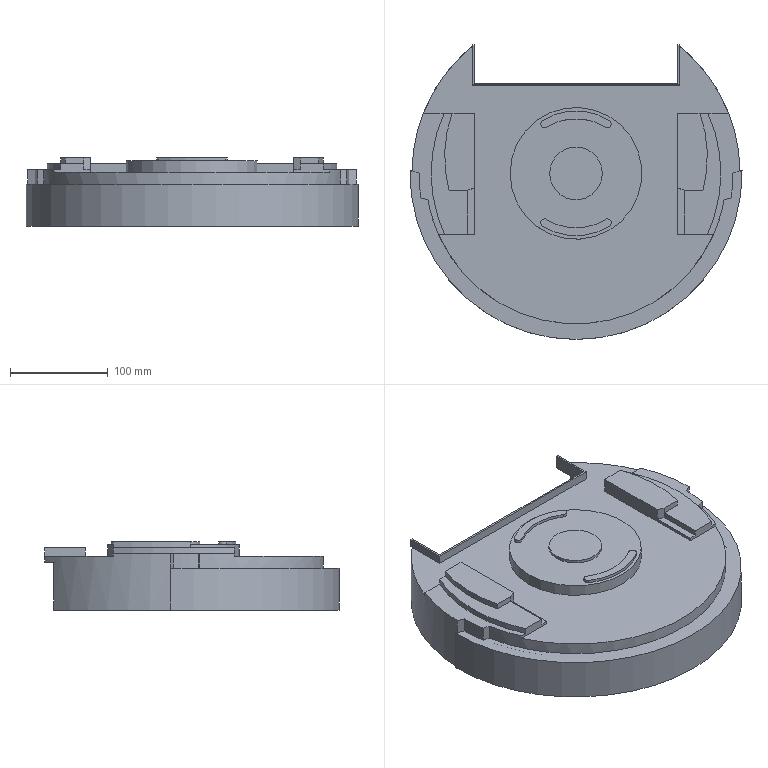Component | NX | INNER_SHELL | 1 solid | 93 faces | volume 2057239 mm3 | plane 68 | cylinder 25 | commonest cylinder face diameters 8.023 x4 336 x2 158.564 x2 321.416 x2 296.678 x2 271.2 x2 112 x2 128 x2